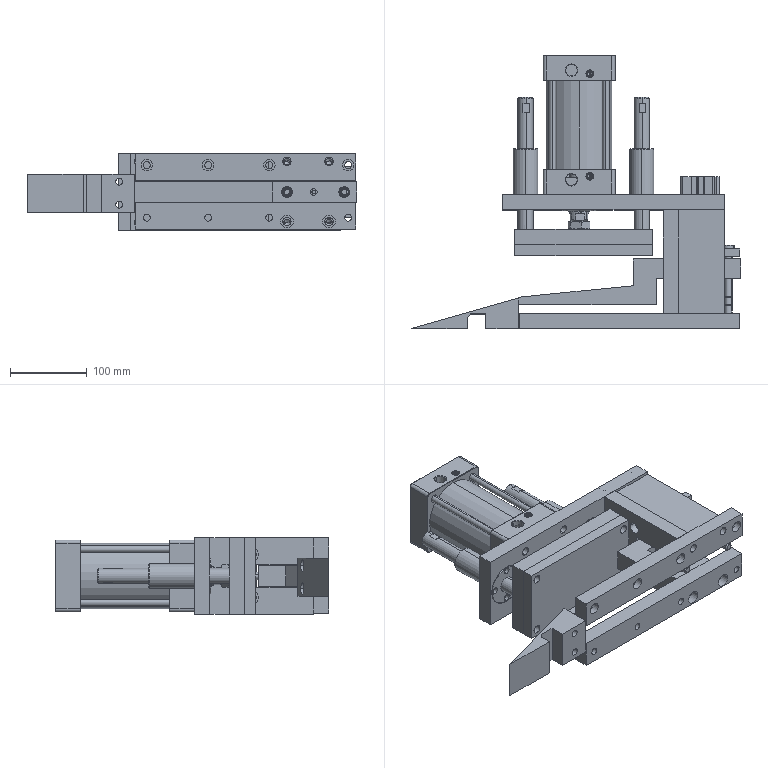Assembly | SolidWorks | mm | 34 component files | 34 solids | 1942 faces | box 430 x 357 x 100 mm | volume 3127936 mm3 | cylinder 711 | plane 688 | cone 357 | spline 150 | torus 36 | commonest cylinder face diameters 10 x64 9 x56 0.4 x46 11 x44 15 x28 8 x27 4.2 x24 16 x23
Bill of materials:
FlangedLinearBearingLMF20L | 2 |  | Flanged cylindrical tube: a long plain cylindrical barrel with a thin circular flange at one end; the flange has four evenly spaced through-holes and the part has a central through-bore.
GA-10-25-2GuideBushing | 2 |  | Flanged sleeve or bushing-like shape: a thin-walled cylindrical tube with a short, larger-diameter collar at one end and a through-bore; the edges are rounded.
GP-10-100-2GuidePin | 2 |  | Headed pin: a long slender cylindrical shank with a short, larger cylindrical head at one end and a chamfered or rounded tip at the other; three narrow circumferential grooves sit near the tip end.
10 | 1 |  | Plain cylindrical tube or spacer: a thick-walled hollow cylinder with a central through-bore and rounded outer end edges.
1 | 1 |  | Housing with a cylindrical barrel between two square end blocks. Each block has four corner through-holes and, on one side face, a larger and a smaller round hole. One end has a protruding cylindrical boss with a bore, and the end face has radial ribs/slots around a central circular feature.
11 | 1 |  | Plain cylindrical tube or spacer: a thick-walled hollow cylinder with a central through-bore and rounded outer end edges.
12 | 1 |  | Stepped cylindrical plug or screw-like part. The top has a hexagonal socket with a conical bottom, and below it are several circumferential grooves with a rounded ring-shaped element in one groove. Below that is a plain cylindrical body, then a narrower stepped and tapered tip.
13 | 1 |  | Stepped cylindrical plug or screw-like part. The top has a hexagonal socket with a conical bottom, and below it are several circumferential grooves with a rounded ring-shaped element in one groove. Below that is a plain cylindrical body, then a narrower stepped and tapered tip.
14 | 1 |  | Thin flat annular ring with six evenly spaced rectangular tabs on its outer edge. The tabs are bent out of the ring plane at various angles (some steeply, some near vertical), giving a tab-washer-like shape.
15 | 1 |  | Thin flat annular ring with six evenly spaced rectangular tabs on its outer edge. The tabs are bent out of the ring plane at various angles (some steeply, some near vertical), giving a tab-washer-like shape.
2 | 1 |  | Stepped shaft carrying a larger disc-shaped hub. The hub's outer surface has several circumferential grooves, and its face has a recessed annular cavity divided by radial ribs. The shaft has several diameter steps and a small flat or notch near the narrow end.
3 | 1 |  | Hexagonal nut-like body: a hexagonal prism with chamfered corners on both faces and a central circular through-bore.
4 | 1 |  | Long slender cylindrical rod with an enlarged cylindrical end section at each end; the larger end has a hexagonal socket recess, and the other end has a shorter, smaller collar.
5 | 1 |  | Long slender cylindrical rod with an enlarged cylindrical end section at each end; the larger end has a hexagonal socket recess, and the other end has a shorter, smaller collar.
6 | 1 |  | Long slender cylindrical rod with an enlarged cylindrical end section at each end; the larger end has a hexagonal socket recess, and the other end has a shorter, smaller collar.
7 | 1 |  | Long slender cylindrical rod with an enlarged cylindrical end section at each end; the larger end has a hexagonal socket recess, and the other end has a shorter, smaller collar.
8 | 1 |  | Short thick-walled hollow cylinder (sleeve or tube) with a central through bore and rounded outer end edges.
9 | 1 |  | Short thick-walled hollow cylinder (sleeve or tube) with a central through bore and rounded outer end edges.
SDAS_32x60_B60_r | 1 | 45 | Stepped cylindrical shaft with a large disc-like flanged head carrying two circumferential grooves; the far end steps down to a smaller-diameter pin with a small transition feature.
SDAS_32x6060_b | 1 | 45 | Prismatic extruded-style block with a near-square cross-section, longitudinal slots and grooves on its faces, four corner through holes, a large central circular feature with a short protruding cylindrical boss and bore at one end, and circular ports on one side face.
SHYTJ-01-03-05 | 1 |  | Flat rectangular plate with four small through holes near its corners.
SHYTJ-01-03-06GuideAxis | 2 |  | Long cylindrical tube or rod with an axial bore at one end and a small groove or flat near the other end.
SHYTJ-01-07-01CylinderMountingPlate | 1 |  | Flat rectangular plate with three large through holes in a row, eight medium holes, small holes around the two outer large holes, and an open rectangular slot at one end that forms two prongs with holes.
SHYTJ-01-07-02ShimPlate | 2 |  | Long rectangular bar with six through holes on one face: four smaller holes and two larger holes, unevenly spaced along its length.
SHYTJ-01-07-03SupportPlate | 1 |  | Rectangular block with a C/U-shaped profile: a solid spine with two parallel flat arms enclosing an open-ended rectangular slot. Several small round holes, one larger round hole in the spine, and a narrow shallow groove along one top edge.
SHYTJ-01-07-04PressurePlate | 1 |  | Flat rectangular plate with three round through holes in a line along its long axis: a larger hole in the center and two smaller holes near the ends.
SHYTJ-01-07-05BlankingBlock1-2 | 1 |  | Long, slender rectangular-section bar with a joggle (offset step) near mid-length. One segment tapers in height toward its free end. The straight segment has two round holes with a much smaller hole between them.
SHYTJ-01-07-06CylinderMountingPlate | 1 |  | Thick rectangular plate with one large round bore, four smaller holes in a rectangular pattern around it, one medium hole off to one side, and a small hole drilled into one edge face.
SHYTJ-01-07-07GuideBlock | 1 |  | Wedge-shaped block, thin at one end and full height at the other, with a rectangular notch cut through its width partway along its length. Two round holes are in the thick end section.
Mates:
1. coincident | SHYTJ-01-07-01CylinderMountingPlate-1 face at (-80.116, -20.361, 320) dir (0, -1, 0) | SHYTJ-01-07-03SupportPlate-1 face at (129.884, -20.361, 220) dir (0, 1, 0)
2. concentric | SHYTJ-01-07-01CylinderMountingPlate-1 face at (139.884, -0.3608, 310) dir (0, 1, 0) r 9 | SHYTJ-01-07-03SupportPlate-1 face at (139.884, -20.361, 310) dir (0, 1, 0) r 4.25
3. concentric | SHYTJ-01-07-01CylinderMountingPlate-1 face at (139.884, -0.3608, 230) dir (0, 1, 0) r 9 | SHYTJ-01-07-03SupportPlate-1 face at (139.884, -20.361, 230) dir (0, 1, 0) r 4.25
4. coincident | SHYTJ-01-07-02ShimPlate-1 face at (-58.116, -155.361, 221.5) dir (0, 1, 0) | SHYTJ-01-07-03SupportPlate-1 face at (129.884, -155.361, 220) dir (0, -1, 0)
5. concentric | SHYTJ-01-07-01CylinderMountingPlate-1 face at (-50.116, -20.361, 270) dir (0, 1, 0) r 16.5 | FlangedLinearBearingLMF20L-1 face at (-50.116, -20.361, 270) dir (0, -1, 0) r 16
6. coincident | SHYTJ-01-07-01CylinderMountingPlate-1 face at (-50.116, -12.361, 270) dir (0, -1, 0) | FlangedLinearBearingLMF20L-1 face at (-77.116, -12.361, 270) dir (0, 1, 0)
7. concentric | SHYTJ-01-07-01CylinderMountingPlate-1 face at (-71.616, -12.361, 270) dir (0, -1, 0) r 2.1 | FlangedLinearBearingLMF20L-1 face at (-71.616, -20.361, 270) dir (0, -1, 0) r 4.5
8. concentric | SHYTJ-01-03-06GuideAxis-1 face at (-50.116, -48.361, 270) dir (0, -1, 0) r 10 | SHYTJ-01-07-04PressurePlate-1 face at (-50.116, -55.361, 270) dir (0, -1, 0) r 8.5
9. coincident | SHYTJ-01-03-06GuideAxis-1 face at (-50.116, -48.361, 270) dir (0, -1, 0) | SHYTJ-01-07-04PressurePlate-1 face at (-50.116, -48.361, 270) dir (0, 1, 0)
10. concentric | SHYTJ-01-03-06GuideAxis-1 face at (-50.116, -48.361, 270) dir (0, -1, 0) r 10 | FlangedLinearBearingLMF20L-1 face at (-50.116, -20.361, 270) dir (0, -1, 0) r 16
11. concentric | SHYTJ-01-07-04PressurePlate-1 face at (101.884, -48.361, 270) dir (0, 1, 0) r 10 | SHYTJ-01-03-06GuideAxis-2 face at (101.884, -48.361, 270) dir (0, -1, 0) r 10
12. coincident | SHYTJ-01-07-04PressurePlate-1 face at (-64.116, -65.361, 320) dir (0, -1, 0) | SHYTJ-01-03-05-1 face at (115.884, -65.361, 220) dir (0, 1, 0)
13. coincident | SHYTJ-01-07-04PressurePlate-1 face at (-64.116, -65.361, 320) dir (0, 0, 1) | SHYTJ-01-03-05-1 face at (115.884, -65.361, 320) dir (0, 0, 1)
14. coincident | SHYTJ-01-07-04PressurePlate-1 face at (115.884, -65.361, 320) dir (1, 0, 0) | SHYTJ-01-03-05-1 face at (115.884, -65.361, 220) dir (1, 0, 0)
15. concentric | SHYTJ-01-07-03SupportPlate-1 face at (139.884, -20.361, 270) dir (0, -1, 0) r 5 | GP-10-100-2GuidePin-2 face at (139.884, -165.161, 270) dir (0, -1, 0) r 5
16. coincident | SHYTJ-01-07-03SupportPlate-1 face at (139.884, -70.361, 270) dir (0, 1, 0) | GP-10-100-2GuidePin-2 face at (144.582, -70.361, 268.288) dir (0, -1, 0)
17. coincident | SHYTJ-01-07-03SupportPlate-1 face at (149.884, -20.361, 220) dir (1, 0, 0) | SHYTJ-01-07-06CylinderMountingPlate-1 face at (149.884, -81.361, 303) dir (-1, 0, 0)
18. coincident | SDAS_32x60_B_0-1/SDAS_32x6060_b-1 face at (183.284, -71.361, 248.2) dir (0, -1, 0) | SHYTJ-01-07-06CylinderMountingPlate-1 face at (174.884, -71.361, 270) dir (0, 1, 0)
19. concentric | SDAS_32x60_B_0-1/SDAS_32x6060_b-1 face at (191.884, -24.111, 287) dir (0, -1, 0) r 4.1 | SHYTJ-01-07-06CylinderMountingPlate-1 face at (191.884, -81.361, 287) dir (0, -1, 0) r 5.5
20. concentric | SDAS_32x60_B_0-1/SDAS_32x6060_b-1 face at (191.884, -24.111, 253) dir (0, -1, 0) r 2.458 | SHYTJ-01-07-06CylinderMountingPlate-1 face at (191.884, -81.361, 253) dir (0, -1, 0) r 5.5
21. concentric | SHYTJ-01-07-03SupportPlate-1 face at (129.884, -76.361, 242) dir (-1, 0, 0) r 4.5 | SHYTJ-01-07-06CylinderMountingPlate-1 face at (149.884, -76.361, 242) dir (-1, 0, 0) r 3.4
22. concentric | SHYTJ-01-07-03SupportPlate-1 face at (129.884, -76.361, 298) dir (-1, 0, 0) r 4.5 | SHYTJ-01-07-06CylinderMountingPlate-1 face at (149.884, -76.361, 298) dir (-1, 0, 0) r 3.4
23. concentric | GP-10-100-2GuidePin-1 face at (214.884, -166.161, 270) dir (0, -1, 0) r 5 | SHYTJ-01-07-06CylinderMountingPlate-1 face at (214.884, -81.361, 270) dir (0, 1, 0) r 5
24. coincident | GP-10-100-2GuidePin-1 face at (210.698, -71.361, 267.265) dir (0, -1, 0) | SHYTJ-01-07-06CylinderMountingPlate-1 face at (174.884, -71.361, 270) dir (0, 1, 0)
25. concentric | GP-10-100-2GuidePin-2 face at (139.884, -165.161, 270) dir (0, -1, 0) r 5 | GA-10-25-2GuideBushing-2 face at (139.884, -84.361, 270) dir (0, 1, 0) r 5
26. concentric | GP-10-100-2GuidePin-1 face at (214.884, -166.161, 270) dir (0, -1, 0) r 5 | GA-10-25-2GuideBushing-1 face at (214.884, -84.361, 270) dir (0, 1, 0) r 5
27. concentric | SHYTJ-01-07-03SupportPlate-1 face at (194.889, -155.361, 310) dir (0, -1, 0) r 4.25 | SHYTJ-01-07-02ShimPlate-3 face at (194.889, -155.361, 310) dir (0, 1, 0) r 8.5
28. concentric | SHYTJ-01-07-03SupportPlate-1 face at (139.889, -155.361, 310) dir (0, -1, 0) r 4.25 | SHYTJ-01-07-02ShimPlate-3 face at (139.889, -155.361, 310) dir (0, 1, 0) r 5.5
29. coincident | SHYTJ-01-07-02ShimPlate-1 face at (-58.116, -175.361, 221.5) dir (0, -1, 0) | SHYTJ-01-07-02ShimPlate-3 face at (-58.111, -175.361, 320) dir (0, -1, 0)
30. parallel | SHYTJ-01-07-02ShimPlate-1 face at (229.884, -175.361, 221.5) dir (1, 0, 0) | SHYTJ-01-07-02ShimPlate-3 face at (229.889, -155.361, 320) dir (1, 0, 0)
31. concentric | GA-10-25-2GuideBushing-1 face at (214.884, -84.361, 270) dir (0, 1, 0) r 7 | SHYTJ-01-07-05BlankingBlock1-2-1 face at (214.884, -144.361, 270) dir (0, 1, 0) r 7
32. concentric | GA-10-25-2GuideBushing-2 face at (139.884, -84.361, 270) dir (0, 1, 0) r 7 | SHYTJ-01-07-05BlankingBlock1-2-1 face at (139.884, -87.361, 270) dir (0, 1, 0) r 9
33. coincident | GA-10-25-2GuideBushing-1 face at (208.501, -87.361, 267.127) dir (0, -1, 0) | SHYTJ-01-07-05BlankingBlock1-2-1 face at (214.884, -87.361, 270) dir (0, 1, 0)
34. coincident | assembly face at (174.884, -84.361, 270) dir (0, -1, 0) | SHYTJ-01-07-05BlankingBlock1-2-1 face at (230.884, -84.361, 256.5) dir (0, 1, 0)
35. concentric | SHYTJ-01-07-01CylinderMountingPlate-1 face at (19.884, -20.361, 270) dir (0, 1, 0) r 24 | SC-80x75(000)-1/1-1 face at (19.884, -0.3608, 270) dir (0, -1, 0) r 23.5
36. coincident | SHYTJ-01-07-04PressurePlate-1 face at (-64.116, -45.361, 320) dir (0, 1, 0) | SC-80x75(000)-1/3-1 face at (21.132, -45.361, 276.379) dir (0, -1, 0)
37. coincident | SHYTJ-01-07-01CylinderMountingPlate-1 face at (209.884, -0.3608, 320) dir (0, 1, 0) | SC-80x75(000)-1/1-1 face at (19.884, -0.3608, 270) dir (0, -1, 0)
38. concentric | SHYTJ-01-07-01CylinderMountingPlate-1 face at (54.884, -20.361, 235) dir (0, -1, 0) r 5.5 | SC-80x75(000)-1/5-1 face at (54.884, 90.639, 235) dir (0, 1, 0) r 4.45
39. concentric | SHYTJ-01-07-01CylinderMountingPlate-1 face at (-15.116, -20.361, 235) dir (0, -1, 0) r 5.5 | SC-80x75(000)-1/7-1 face at (-15.116, 90.639, 235) dir (0, 1, 0) r 4.45
40. lock | 1-1 reference at (0, 0, 0) dir (1, 0, 0) | 6-1 reference at (0, 0, 0) dir (1, 0, 0)
41. lock | 1-1 reference at (0, 0, 0) dir (1, 0, 0) | 7-1 reference at (0, 0, 0) dir (1, 0, 0)
42. lock | 1-1 reference at (0, 0, 0) dir (1, 0, 0) | 5-1 reference at (0, 0, 0) dir (1, 0, 0)
43. lock | 1-1 reference at (0, 0, 0) dir (1, 0, 0) | 4-1 reference at (0, 0, 0) dir (1, 0, 0)
44. concentric | 1-1 face at (0, 0, 0) dir (-1, 0, 0) r 23.5 | 2-1 face at (-54.54, 0, 0) dir (1, 0, 0) r 10
45. concentric | 2-1 face at (-54.54, 0, 0) dir (1, 0, 0) r 10 | 3-1 face at (-40, 0, 0) dir (1, 0, 0) r 9.188
46. distance | 3-1 face at (-45, -1.247, 6.379) dir (-1, 0, 0) | 2-1 face at (-60, -102.821, -66.772) dir (-1, 0, 0)
47. distance | 2-1 face at (143, -21.984, -27.931) dir (1, 0, 0) | 1-1 face at (143, 29.1, 0) dir (-1, 0, 0)
48. coincident | SDAS_32x6060_b-1 axis at (-80.9, 0, 0) dir (1, 0, 0) | SDAS_32x60_B60_r-1 axis at (80.9, 0, 0) dir (-1, 0, 0)
49. coincident | SDAS_32x6060_b-1 axis at (-80.9, 0, 0) dir (1, 0, 0) | SDAS_32x60_B60_r-1 axis at (80.9, 0, 0) dir (-1, 0, 0)
50. angle | SDAS_32x60_B60_r-1 plane at (0, 0, 0) dir (0, 0, -1) | SDAS_32x6060_b-1 plane at (0, 0, 0) dir (0, 1, 0)
51. distance | SDAS_32x60_B60_r-1 face at (88.5, 14.15, 0) dir (1, 0, 0) | SDAS_32x6060_b-1 face at (88.5, 0, 16) dir (-1, 0, 0)